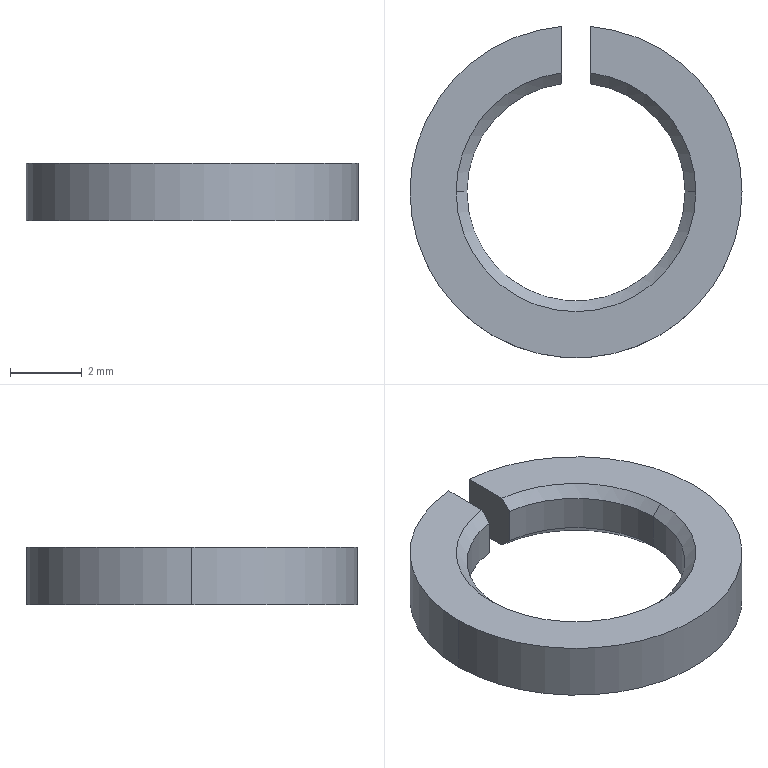Component | SolidWorks | StandardTypeSpringWasher(Assembly)6_1.6[GB_T93-1987]-1 | 1 solid | 16 faces | box 9.28 x 9.26 x 1.6 mm | volume 58 mm3 | cone 6 | cylinder 6 | plane 4 | commonest cylinder face diameters 6.1 x3 9.282 x3
build123d program:
from build123d import *

# Parameters (mm, degrees)
EXTRUDE1_DEPTH = 1.6
CHAMFER1_SIZE  = 0.3


with BuildPart() as part:
    # Sketch1 → Extrude1 (new body)
    with BuildSketch(Plane.XY):
        with BuildLine():
            Line((-0.4, 4.624), (-0.4, 3.024))
            ThreePointArc((-0.4, 3.024), (0, -3.05), (0.4, 3.024))
            Line((0.4, 3.024), (0.4, 4.624))
            ThreePointArc((0.4, 4.624), (0, -4.641), (-0.4, 4.624))
        make_face()
    extrude(amount=EXTRUDE1_DEPTH)

    # Chamfer1
    chamfer1_edges = [part.edges().sort_by_distance(p)[0] for p in [
        (0, -3.05, 1.6),
        (0, -3.05, 0),
    ]]
    chamfer(chamfer1_edges, length=CHAMFER1_SIZE)


solid = part.part

# Placed as in the assembly
solid = solid.moved(Location((120.494, 22.5, 19.6), (0, 0, 0)))
STEP:
#1=COLOUR_RGB('',0.7922,0.8196,0.9333);
#2=FILL_AREA_STYLE_COLOUR('',#1);
#3=FILL_AREA_STYLE('',(#2));
#4=SURFACE_STYLE_FILL_AREA(#3);
#5=SURFACE_SIDE_STYLE('',(#4));
#6=SURFACE_STYLE_USAGE(.BOTH.,#5);
#7=PRESENTATION_STYLE_ASSIGNMENT((#6));
#8=CARTESIAN_POINT('',(4.864,0.8858,0.7835));
#9=VERTEX_POINT('',#8);
#10=CARTESIAN_POINT('',(4.624,0.8858,0.7835));
#11=VERTEX_POINT('',#10);
#12=CARTESIAN_POINT('',(4.744,0.8858,0.7835));
#13=DIRECTION('',(0.,0.,-1.));
#14=DIRECTION('',(1.,0.,0.));
#15=AXIS2_PLACEMENT_3D('',#12,#13,#14);
#16=CIRCLE('',#15,0.1201);
#17=EDGE_CURVE('',#9,#11,#16,.T.);
#18=ORIENTED_EDGE('',*,*,#17,.F.);
#19=CARTESIAN_POINT('',(4.876,0.8858,0.7717));
#20=VERTEX_POINT('',#19);
#21=CARTESIAN_POINT('',(4.864,0.8858,0.7835));
#22=DIRECTION('',(0.7071,0.,-0.7071));
#23=VECTOR('',#22,39.37);
#24=LINE('',#21,#23);
#25=EDGE_CURVE('',#9,#20,#24,.T.);
#26=ORIENTED_EDGE('',*,*,#25,.T.);
#27=CARTESIAN_POINT('',(4.612,0.8858,0.7717));
#28=VERTEX_POINT('',#27);
#29=CARTESIAN_POINT('',(4.744,0.8858,0.7717));
#30=DIRECTION('',(0.,0.,1.));
#31=DIRECTION('',(1.,0.,0.));
#32=AXIS2_PLACEMENT_3D('',#29,#30,#31);
#33=CIRCLE('',#32,0.1319);
#34=EDGE_CURVE('',#28,#20,#33,.T.);
#35=ORIENTED_EDGE('',*,*,#34,.F.);
#36=CARTESIAN_POINT('',(4.624,0.8858,0.7835));
#37=DIRECTION('',(-0.7071,0.,-0.7071));
#38=VECTOR('',#37,39.37);
#39=LINE('',#36,#38);
#40=EDGE_CURVE('',#11,#28,#39,.T.);
#41=ORIENTED_EDGE('',*,*,#40,.F.);
#42=EDGE_LOOP('',(#18,#26,#35,#41));
#43=FACE_OUTER_BOUND('',#42,.T.);
#44=CARTESIAN_POINT('',(4.744,0.8858,0.7835));
#45=DIRECTION('',(0.,0.,-1.));
#46=DIRECTION('',(-1.,0.,0.));
#47=AXIS2_PLACEMENT_3D('',#44,#45,#46);
#48=CONICAL_SURFACE('',#47,0.1201,0.7854);
#49=ADVANCED_FACE('',(#43),#48,.F.);
#50=CARTESIAN_POINT('',(4.728,1.005,0.7835));
#51=VERTEX_POINT('',#50);
#52=CARTESIAN_POINT('',(4.744,0.8858,0.7835));
#53=DIRECTION('',(0.,0.,-1.));
#54=DIRECTION('',(1.,0.,0.));
#55=AXIS2_PLACEMENT_3D('',#52,#53,#54);
#56=CIRCLE('',#55,0.1201);
#57=EDGE_CURVE('',#11,#51,#56,.T.);
#58=ORIENTED_EDGE('',*,*,#57,.F.);
#59=ORIENTED_EDGE('',*,*,#40,.T.);
#60=CARTESIAN_POINT('',(4.728,1.017,0.7717));
#61=VERTEX_POINT('',#60);
#62=CARTESIAN_POINT('',(4.744,0.8858,0.7717));
#63=DIRECTION('',(0.,0.,1.));
#64=DIRECTION('',(1.,0.,0.));
#65=AXIS2_PLACEMENT_3D('',#62,#63,#64);
#66=CIRCLE('',#65,0.1319);
#67=EDGE_CURVE('',#61,#28,#66,.T.);
#68=ORIENTED_EDGE('',*,*,#67,.F.);
#69=CARTESIAN_POINT('',(4.728,1.005,0.7835));
#70=CARTESIAN_POINT('',(4.728,1.009,0.7795));
#71=CARTESIAN_POINT('',(4.728,1.013,0.7756));
#72=CARTESIAN_POINT('',(4.728,1.017,0.7717));
#73=B_SPLINE_CURVE_WITH_KNOTS('',3,(#69,#70,#71,#72),.UNSPECIFIED.,.F.,.F.,(4,4),(0.,0.0004259),.UNSPECIFIED.);
#74=EDGE_CURVE('',#51,#61,#73,.T.);
#75=ORIENTED_EDGE('',*,*,#74,.F.);
#76=EDGE_LOOP('',(#58,#59,#68,#75));
#77=FACE_OUTER_BOUND('',#76,.T.);
#78=CARTESIAN_POINT('',(4.744,0.8858,0.7835));
#79=DIRECTION('',(0.,0.,-1.));
#80=DIRECTION('',(-1.,0.,0.));
#81=AXIS2_PLACEMENT_3D('',#78,#79,#80);
#82=CONICAL_SURFACE('',#81,0.1201,0.7854);
#83=ADVANCED_FACE('',(#77),#82,.F.);
#84=CARTESIAN_POINT('',(4.624,0.8858,0.8228));
#85=VERTEX_POINT('',#84);
#86=CARTESIAN_POINT('',(4.864,0.8858,0.8228));
#87=VERTEX_POINT('',#86);
#88=CARTESIAN_POINT('',(4.744,0.8858,0.8228));
#89=DIRECTION('',(0.,0.,1.));
#90=DIRECTION('',(1.,0.,0.));
#91=AXIS2_PLACEMENT_3D('',#88,#89,#90);
#92=CIRCLE('',#91,0.1201);
#93=EDGE_CURVE('',#85,#87,#92,.T.);
#94=ORIENTED_EDGE('',*,*,#93,.F.);
#95=CARTESIAN_POINT('',(4.612,0.8858,0.8346));
#96=VERTEX_POINT('',#95);
#97=CARTESIAN_POINT('',(4.612,0.8858,0.8346));
#98=DIRECTION('',(-0.7071,0.,0.7071));
#99=VECTOR('',#98,39.37);
#100=LINE('',#97,#99);
#101=EDGE_CURVE('',#85,#96,#100,.T.);
#102=ORIENTED_EDGE('',*,*,#101,.T.);
#103=CARTESIAN_POINT('',(4.876,0.8858,0.8346));
#104=VERTEX_POINT('',#103);
#105=CARTESIAN_POINT('',(4.744,0.8858,0.8346));
#106=DIRECTION('',(0.,0.,-1.));
#107=DIRECTION('',(1.,0.,0.));
#108=AXIS2_PLACEMENT_3D('',#105,#106,#107);
#109=CIRCLE('',#108,0.1319);
#110=EDGE_CURVE('',#104,#96,#109,.T.);
#111=ORIENTED_EDGE('',*,*,#110,.F.);
#112=CARTESIAN_POINT('',(4.876,0.8858,0.8346));
#113=DIRECTION('',(0.7071,0.,0.7071));
#114=VECTOR('',#113,39.37);
#115=LINE('',#112,#114);
#116=EDGE_CURVE('',#87,#104,#115,.T.);
#117=ORIENTED_EDGE('',*,*,#116,.F.);
#118=EDGE_LOOP('',(#94,#102,#111,#117));
#119=FACE_OUTER_BOUND('',#118,.T.);
#120=CARTESIAN_POINT('',(4.744,0.8858,0.8346));
#121=DIRECTION('',(0.,0.,1.));
#122=DIRECTION('',(1.,0.,0.));
#123=AXIS2_PLACEMENT_3D('',#120,#121,#122);
#124=CONICAL_SURFACE('',#123,0.1319,0.7854);
#125=ADVANCED_FACE('',(#119),#124,.F.);
#126=CARTESIAN_POINT('',(4.76,1.005,0.8228));
#127=VERTEX_POINT('',#126);
#128=CARTESIAN_POINT('',(4.744,0.8858,0.8228));
#129=DIRECTION('',(0.,0.,1.));
#130=DIRECTION('',(1.,0.,0.));
#131=AXIS2_PLACEMENT_3D('',#128,#129,#130);
#132=CIRCLE('',#131,0.1201);
#133=EDGE_CURVE('',#87,#127,#132,.T.);
#134=ORIENTED_EDGE('',*,*,#133,.F.);
#135=ORIENTED_EDGE('',*,*,#116,.T.);
#136=CARTESIAN_POINT('',(4.76,1.017,0.8346));
#137=VERTEX_POINT('',#136);
#138=CARTESIAN_POINT('',(4.744,0.8858,0.8346));
#139=DIRECTION('',(0.,0.,-1.));
#140=DIRECTION('',(1.,0.,0.));
#141=AXIS2_PLACEMENT_3D('',#138,#139,#140);
#142=CIRCLE('',#141,0.1319);
#143=EDGE_CURVE('',#137,#104,#142,.T.);
#144=ORIENTED_EDGE('',*,*,#143,.F.);
#145=CARTESIAN_POINT('',(4.76,1.005,0.8228));
#146=CARTESIAN_POINT('',(4.76,1.009,0.8268));
#147=CARTESIAN_POINT('',(4.76,1.013,0.8307));
#148=CARTESIAN_POINT('',(4.76,1.017,0.8346));
#149=B_SPLINE_CURVE_WITH_KNOTS('',3,(#145,#146,#147,#148),.UNSPECIFIED.,.F.,.F.,(4,4),(0.,0.0004259),.UNSPECIFIED.);
#150=EDGE_CURVE('',#127,#137,#149,.T.);
#151=ORIENTED_EDGE('',*,*,#150,.F.);
#152=EDGE_LOOP('',(#134,#135,#144,#151));
#153=FACE_OUTER_BOUND('',#152,.T.);
#154=CARTESIAN_POINT('',(4.744,0.8858,0.8346));
#155=DIRECTION('',(0.,0.,1.));
#156=DIRECTION('',(1.,0.,0.));
#157=AXIS2_PLACEMENT_3D('',#154,#155,#156);
#158=CONICAL_SURFACE('',#157,0.1319,0.7854);
#159=ADVANCED_FACE('',(#153),#158,.F.);
#160=ORIENTED_EDGE('',*,*,#93,.T.);
#161=CARTESIAN_POINT('',(4.864,0.8858,0.8346));
#162=DIRECTION('',(0.,0.,-1.));
#163=VECTOR('',#162,39.37);
#164=LINE('',#161,#163);
#165=EDGE_CURVE('',#87,#9,#164,.T.);
#166=ORIENTED_EDGE('',*,*,#165,.T.);
#167=ORIENTED_EDGE('',*,*,#17,.T.);
#168=CARTESIAN_POINT('',(4.624,0.8858,0.8346));
#169=DIRECTION('',(0.,0.,-1.));
#170=VECTOR('',#169,39.37);
#171=LINE('',#168,#170);
#172=EDGE_CURVE('',#85,#11,#171,.T.);
#173=ORIENTED_EDGE('',*,*,#172,.F.);
#174=EDGE_LOOP('',(#160,#166,#167,#173));
#175=FACE_OUTER_BOUND('',#174,.T.);
#176=CARTESIAN_POINT('',(4.744,0.8858,0.8346));
#177=DIRECTION('',(0.,0.,-1.));
#178=DIRECTION('',(-1.,0.,0.));
#179=AXIS2_PLACEMENT_3D('',#176,#177,#178);
#180=CYLINDRICAL_SURFACE('',#179,0.1201);
#181=ADVANCED_FACE('',(#175),#180,.F.);
#182=CARTESIAN_POINT('',(4.728,1.005,0.8228));
#183=VERTEX_POINT('',#182);
#184=CARTESIAN_POINT('',(4.744,0.8858,0.8228));
#185=DIRECTION('',(0.,0.,1.));
#186=DIRECTION('',(1.,0.,0.));
#187=AXIS2_PLACEMENT_3D('',#184,#185,#186);
#188=CIRCLE('',#187,0.1201);
#189=EDGE_CURVE('',#183,#85,#188,.T.);
#190=ORIENTED_EDGE('',*,*,#189,.T.);
#191=ORIENTED_EDGE('',*,*,#172,.T.);
#192=ORIENTED_EDGE('',*,*,#57,.T.);
#193=CARTESIAN_POINT('',(4.728,1.005,0.8346));
#194=DIRECTION('',(0.,0.,-1.));
#195=VECTOR('',#194,39.37);
#196=LINE('',#193,#195);
#197=EDGE_CURVE('',#183,#51,#196,.T.);
#198=ORIENTED_EDGE('',*,*,#197,.F.);
#199=EDGE_LOOP('',(#190,#191,#192,#198));
#200=FACE_OUTER_BOUND('',#199,.T.);
#201=CARTESIAN_POINT('',(4.744,0.8858,0.8346));
#202=DIRECTION('',(0.,0.,-1.));
#203=DIRECTION('',(-1.,0.,0.));
#204=AXIS2_PLACEMENT_3D('',#201,#202,#203);
#205=CYLINDRICAL_SURFACE('',#204,0.1201);
#206=ADVANCED_FACE('',(#200),#205,.F.);
#207=CARTESIAN_POINT('',(4.927,0.8858,0.8346));
#208=VERTEX_POINT('',#207);
#209=CARTESIAN_POINT('',(4.76,1.068,0.8346));
#210=VERTEX_POINT('',#209);
#211=CARTESIAN_POINT('',(4.744,0.8858,0.8346));
#212=DIRECTION('',(0.,0.,1.));
#213=DIRECTION('',(1.,0.,0.));
#214=AXIS2_PLACEMENT_3D('',#211,#212,#213);
#215=CIRCLE('',#214,0.1827);
#216=EDGE_CURVE('',#208,#210,#215,.T.);
#217=ORIENTED_EDGE('',*,*,#216,.F.);
#218=CARTESIAN_POINT('',(4.927,0.8858,0.7717));
#219=VERTEX_POINT('',#218);
#220=CARTESIAN_POINT('',(4.927,0.8858,0.8346));
#221=DIRECTION('',(0.,0.,-1.));
#222=VECTOR('',#221,39.37);
#223=LINE('',#220,#222);
#224=EDGE_CURVE('',#208,#219,#223,.T.);
#225=ORIENTED_EDGE('',*,*,#224,.T.);
#226=CARTESIAN_POINT('',(4.76,1.068,0.7717));
#227=VERTEX_POINT('',#226);
#228=CARTESIAN_POINT('',(4.744,0.8858,0.7717));
#229=DIRECTION('',(0.,0.,1.));
#230=DIRECTION('',(1.,0.,0.));
#231=AXIS2_PLACEMENT_3D('',#228,#229,#230);
#232=CIRCLE('',#231,0.1827);
#233=EDGE_CURVE('',#219,#227,#232,.T.);
#234=ORIENTED_EDGE('',*,*,#233,.T.);
#235=CARTESIAN_POINT('',(4.76,1.068,0.8346));
#236=DIRECTION('',(0.,0.,-1.));
#237=VECTOR('',#236,39.37);
#238=LINE('',#235,#237);
#239=EDGE_CURVE('',#210,#227,#238,.T.);
#240=ORIENTED_EDGE('',*,*,#239,.F.);
#241=EDGE_LOOP('',(#217,#225,#234,#240));
#242=FACE_OUTER_BOUND('',#241,.T.);
#243=CARTESIAN_POINT('',(4.744,0.8858,0.8346));
#244=DIRECTION('',(0.,0.,-1.));
#245=DIRECTION('',(-1.,0.,0.));
#246=AXIS2_PLACEMENT_3D('',#243,#244,#245);
#247=CYLINDRICAL_SURFACE('',#246,0.1827);
#248=ADVANCED_FACE('',(#242),#247,.T.);
#249=ORIENTED_EDGE('',*,*,#224,.F.);
#250=CARTESIAN_POINT('',(4.561,0.8858,0.8346));
#251=VERTEX_POINT('',#250);
#252=CARTESIAN_POINT('',(4.744,0.8858,0.8346));
#253=DIRECTION('',(0.,0.,1.));
#254=DIRECTION('',(1.,0.,0.));
#255=AXIS2_PLACEMENT_3D('',#252,#253,#254);
#256=CIRCLE('',#255,0.1827);
#257=EDGE_CURVE('',#251,#208,#256,.T.);
#258=ORIENTED_EDGE('',*,*,#257,.F.);
#259=CARTESIAN_POINT('',(4.561,0.8858,0.7717));
#260=VERTEX_POINT('',#259);
#261=CARTESIAN_POINT('',(4.561,0.8858,0.8346));
#262=DIRECTION('',(0.,0.,-1.));
#263=VECTOR('',#262,39.37);
#264=LINE('',#261,#263);
#265=EDGE_CURVE('',#251,#260,#264,.T.);
#266=ORIENTED_EDGE('',*,*,#265,.T.);
#267=CARTESIAN_POINT('',(4.744,0.8858,0.7717));
#268=DIRECTION('',(0.,0.,1.));
#269=DIRECTION('',(1.,0.,0.));
#270=AXIS2_PLACEMENT_3D('',#267,#268,#269);
#271=CIRCLE('',#270,0.1827);
#272=EDGE_CURVE('',#260,#219,#271,.T.);
#273=ORIENTED_EDGE('',*,*,#272,.T.);
#274=EDGE_LOOP('',(#249,#258,#266,#273));
#275=FACE_OUTER_BOUND('',#274,.T.);
#276=CARTESIAN_POINT('',(4.744,0.8858,0.8346));
#277=DIRECTION('',(0.,0.,-1.));
#278=DIRECTION('',(-1.,0.,0.));
#279=AXIS2_PLACEMENT_3D('',#276,#277,#278);
#280=CYLINDRICAL_SURFACE('',#279,0.1827);
#281=ADVANCED_FACE('',(#275),#280,.T.);
#282=ORIENTED_EDGE('',*,*,#265,.F.);
#283=CARTESIAN_POINT('',(4.728,1.068,0.8346));
#284=VERTEX_POINT('',#283);
#285=CARTESIAN_POINT('',(4.744,0.8858,0.8346));
#286=DIRECTION('',(0.,0.,1.));
#287=DIRECTION('',(1.,0.,0.));
#288=AXIS2_PLACEMENT_3D('',#285,#286,#287);
#289=CIRCLE('',#288,0.1827);
#290=EDGE_CURVE('',#284,#251,#289,.T.);
#291=ORIENTED_EDGE('',*,*,#290,.F.);
#292=CARTESIAN_POINT('',(4.728,1.068,0.7717));
#293=VERTEX_POINT('',#292);
#294=CARTESIAN_POINT('',(4.728,1.068,0.8346));
#295=DIRECTION('',(0.,0.,-1.));
#296=VECTOR('',#295,39.37);
#297=LINE('',#294,#296);
#298=EDGE_CURVE('',#284,#293,#297,.T.);
#299=ORIENTED_EDGE('',*,*,#298,.T.);
#300=CARTESIAN_POINT('',(4.744,0.8858,0.7717));
#301=DIRECTION('',(0.,0.,1.));
#302=DIRECTION('',(1.,0.,0.));
#303=AXIS2_PLACEMENT_3D('',#300,#301,#302);
#304=CIRCLE('',#303,0.1827);
#305=EDGE_CURVE('',#293,#260,#304,.T.);
#306=ORIENTED_EDGE('',*,*,#305,.T.);
#307=EDGE_LOOP('',(#282,#291,#299,#306));
#308=FACE_OUTER_BOUND('',#307,.T.);
#309=CARTESIAN_POINT('',(4.744,0.8858,0.8346));
#310=DIRECTION('',(0.,0.,-1.));
#311=DIRECTION('',(-1.,0.,0.));
#312=AXIS2_PLACEMENT_3D('',#309,#310,#311);
#313=CYLINDRICAL_SURFACE('',#312,0.1827);
#314=ADVANCED_FACE('',(#308),#313,.T.);
#315=CARTESIAN_POINT('',(4.76,1.005,0.7835));
#316=VERTEX_POINT('',#315);
#317=CARTESIAN_POINT('',(4.76,1.005,0.8346));
#318=DIRECTION('',(0.,0.,-1.));
#319=VECTOR('',#318,39.37);
#320=LINE('',#317,#319);
#321=EDGE_CURVE('',#127,#316,#320,.T.);
#322=ORIENTED_EDGE('',*,*,#321,.F.);
#323=ORIENTED_EDGE('',*,*,#150,.T.);
#324=CARTESIAN_POINT('',(4.76,1.068,0.8346));
#325=DIRECTION('',(0.,-1.,0.));
#326=VECTOR('',#325,39.37);
#327=LINE('',#324,#326);
#328=EDGE_CURVE('',#210,#137,#327,.T.);
#329=ORIENTED_EDGE('',*,*,#328,.F.);
#330=ORIENTED_EDGE('',*,*,#239,.T.);
#331=CARTESIAN_POINT('',(4.76,1.017,0.7717));
#332=VERTEX_POINT('',#331);
#333=CARTESIAN_POINT('',(4.76,1.068,0.7717));
#334=DIRECTION('',(0.,-1.,0.));
#335=VECTOR('',#334,39.37);
#336=LINE('',#333,#335);
#337=EDGE_CURVE('',#227,#332,#336,.T.);
#338=ORIENTED_EDGE('',*,*,#337,.T.);
#339=CARTESIAN_POINT('',(4.76,1.017,0.7717));
#340=CARTESIAN_POINT('',(4.76,1.013,0.7756));
#341=CARTESIAN_POINT('',(4.76,1.009,0.7795));
#342=CARTESIAN_POINT('',(4.76,1.005,0.7835));
#343=B_SPLINE_CURVE_WITH_KNOTS('',3,(#339,#340,#341,#342),.UNSPECIFIED.,.F.,.F.,(4,4),(0.,0.0004259),.UNSPECIFIED.);
#344=EDGE_CURVE('',#332,#316,#343,.T.);
#345=ORIENTED_EDGE('',*,*,#344,.T.);
#346=EDGE_LOOP('',(#322,#323,#329,#330,#338,#345));
#347=FACE_OUTER_BOUND('',#346,.T.);
#348=CARTESIAN_POINT('',(4.76,1.068,0.8346));
#349=DIRECTION('',(1.,0.,0.));
#350=DIRECTION('',(-0.,1.,0.));
#351=AXIS2_PLACEMENT_3D('',#348,#349,#350);
#352=PLANE('',#351);
#353=ADVANCED_FACE('',(#347),#352,.F.);
#354=ORIENTED_EDGE('',*,*,#165,.F.);
#355=ORIENTED_EDGE('',*,*,#133,.T.);
#356=ORIENTED_EDGE('',*,*,#321,.T.);
#357=CARTESIAN_POINT('',(4.744,0.8858,0.7835));
#358=DIRECTION('',(0.,0.,-1.));
#359=DIRECTION('',(1.,0.,0.));
#360=AXIS2_PLACEMENT_3D('',#357,#358,#359);
#361=CIRCLE('',#360,0.1201);
#362=EDGE_CURVE('',#316,#9,#361,.T.);
#363=ORIENTED_EDGE('',*,*,#362,.T.);
#364=EDGE_LOOP('',(#354,#355,#356,#363));
#365=FACE_OUTER_BOUND('',#364,.T.);
#366=CARTESIAN_POINT('',(4.744,0.8858,0.8346));
#367=DIRECTION('',(0.,0.,-1.));
#368=DIRECTION('',(-1.,0.,0.));
#369=AXIS2_PLACEMENT_3D('',#366,#367,#368);
#370=CYLINDRICAL_SURFACE('',#369,0.1201);
#371=ADVANCED_FACE('',(#365),#370,.F.);
#372=CARTESIAN_POINT('',(4.728,1.017,0.8346));
#373=VERTEX_POINT('',#372);
#374=CARTESIAN_POINT('',(4.728,1.068,0.8346));
#375=DIRECTION('',(0.,1.,0.));
#376=VECTOR('',#375,39.37);
#377=LINE('',#374,#376);
#378=EDGE_CURVE('',#373,#284,#377,.T.);
#379=ORIENTED_EDGE('',*,*,#378,.F.);
#380=CARTESIAN_POINT('',(4.728,1.017,0.8346));
#381=CARTESIAN_POINT('',(4.728,1.013,0.8307));
#382=CARTESIAN_POINT('',(4.728,1.009,0.8268));
#383=CARTESIAN_POINT('',(4.728,1.005,0.8228));
#384=B_SPLINE_CURVE_WITH_KNOTS('',3,(#380,#381,#382,#383),.UNSPECIFIED.,.F.,.F.,(4,4),(0.,0.0004259),.UNSPECIFIED.);
#385=EDGE_CURVE('',#373,#183,#384,.T.);
#386=ORIENTED_EDGE('',*,*,#385,.T.);
#387=ORIENTED_EDGE('',*,*,#197,.T.);
#388=ORIENTED_EDGE('',*,*,#74,.T.);
#389=CARTESIAN_POINT('',(4.728,1.068,0.7717));
#390=DIRECTION('',(0.,1.,0.));
#391=VECTOR('',#390,39.37);
#392=LINE('',#389,#391);
#393=EDGE_CURVE('',#61,#293,#392,.T.);
#394=ORIENTED_EDGE('',*,*,#393,.T.);
#395=ORIENTED_EDGE('',*,*,#298,.F.);
#396=EDGE_LOOP('',(#379,#386,#387,#388,#394,#395));
#397=FACE_OUTER_BOUND('',#396,.T.);
#398=CARTESIAN_POINT('',(4.728,1.068,0.8346));
#399=DIRECTION('',(-1.,0.,0.));
#400=DIRECTION('',(0.,0.,1.));
#401=AXIS2_PLACEMENT_3D('',#398,#399,#400);
#402=PLANE('',#401);
#403=ADVANCED_FACE('',(#397),#402,.F.);
#404=ORIENTED_EDGE('',*,*,#328,.T.);
#405=ORIENTED_EDGE('',*,*,#143,.T.);
#406=ORIENTED_EDGE('',*,*,#110,.T.);
#407=CARTESIAN_POINT('',(4.744,0.8858,0.8346));
#408=DIRECTION('',(0.,0.,-1.));
#409=DIRECTION('',(1.,0.,0.));
#410=AXIS2_PLACEMENT_3D('',#407,#408,#409);
#411=CIRCLE('',#410,0.1319);
#412=EDGE_CURVE('',#96,#373,#411,.T.);
#413=ORIENTED_EDGE('',*,*,#412,.T.);
#414=ORIENTED_EDGE('',*,*,#378,.T.);
#415=ORIENTED_EDGE('',*,*,#290,.T.);
#416=ORIENTED_EDGE('',*,*,#257,.T.);
#417=ORIENTED_EDGE('',*,*,#216,.T.);
#418=EDGE_LOOP('',(#404,#405,#406,#413,#414,#415,#416,#417));
#419=FACE_OUTER_BOUND('',#418,.T.);
#420=CARTESIAN_POINT('',(4.744,0.8858,0.8346));
#421=DIRECTION('',(0.,0.,1.));
#422=DIRECTION('',(1.,0.,0.));
#423=AXIS2_PLACEMENT_3D('',#420,#421,#422);
#424=PLANE('',#423);
#425=ADVANCED_FACE('',(#419),#424,.T.);
#426=ORIENTED_EDGE('',*,*,#393,.F.);
#427=ORIENTED_EDGE('',*,*,#67,.T.);
#428=ORIENTED_EDGE('',*,*,#34,.T.);
#429=CARTESIAN_POINT('',(4.744,0.8858,0.7717));
#430=DIRECTION('',(0.,0.,1.));
#431=DIRECTION('',(1.,0.,0.));
#432=AXIS2_PLACEMENT_3D('',#429,#430,#431);
#433=CIRCLE('',#432,0.1319);
#434=EDGE_CURVE('',#20,#332,#433,.T.);
#435=ORIENTED_EDGE('',*,*,#434,.T.);
#436=ORIENTED_EDGE('',*,*,#337,.F.);
#437=ORIENTED_EDGE('',*,*,#233,.F.);
#438=ORIENTED_EDGE('',*,*,#272,.F.);
#439=ORIENTED_EDGE('',*,*,#305,.F.);
#440=EDGE_LOOP('',(#426,#427,#428,#435,#436,#437,#438,#439));
#441=FACE_OUTER_BOUND('',#440,.T.);
#442=CARTESIAN_POINT('',(4.744,0.8858,0.7717));
#443=DIRECTION('',(0.,0.,1.));
#444=DIRECTION('',(1.,0.,0.));
#445=AXIS2_PLACEMENT_3D('',#442,#443,#444);
#446=PLANE('',#445);
#447=ADVANCED_FACE('',(#441),#446,.F.);
#448=ORIENTED_EDGE('',*,*,#101,.F.);
#449=ORIENTED_EDGE('',*,*,#189,.F.);
#450=ORIENTED_EDGE('',*,*,#385,.F.);
#451=ORIENTED_EDGE('',*,*,#412,.F.);
#452=EDGE_LOOP('',(#448,#449,#450,#451));
#453=FACE_OUTER_BOUND('',#452,.T.);
#454=CARTESIAN_POINT('',(4.744,0.8858,0.8346));
#455=DIRECTION('',(0.,0.,1.));
#456=DIRECTION('',(1.,0.,0.));
#457=AXIS2_PLACEMENT_3D('',#454,#455,#456);
#458=CONICAL_SURFACE('',#457,0.1319,0.7854);
#459=ADVANCED_FACE('',(#453),#458,.F.);
#460=ORIENTED_EDGE('',*,*,#25,.F.);
#461=ORIENTED_EDGE('',*,*,#362,.F.);
#462=ORIENTED_EDGE('',*,*,#344,.F.);
#463=ORIENTED_EDGE('',*,*,#434,.F.);
#464=EDGE_LOOP('',(#460,#461,#462,#463));
#465=FACE_OUTER_BOUND('',#464,.T.);
#466=CARTESIAN_POINT('',(4.744,0.8858,0.7835));
#467=DIRECTION('',(0.,0.,-1.));
#468=DIRECTION('',(-1.,0.,0.));
#469=AXIS2_PLACEMENT_3D('',#466,#467,#468);
#470=CONICAL_SURFACE('',#469,0.1201,0.7854);
#471=ADVANCED_FACE('',(#465),#470,.F.);
#472=CLOSED_SHELL('',(#49,#83,#125,#159,#181,#206,#248,#281,#314,#353,#371,#403,#425,#447,#459,#471));
#473=MANIFOLD_SOLID_BREP('',#472);
#474=STYLED_ITEM('',(#7),#473);
#475=PRESENTATION_LAYER_ASSIGNMENT('','',(#474));
#476=(LENGTH_UNIT()NAMED_UNIT(*)SI_UNIT($,.METRE.));
#477=LENGTH_MEASURE_WITH_UNIT(LENGTH_MEASURE(0.0254),#476);
#478=DIMENSIONAL_EXPONENTS(1.,0.,0.,0.,0.,0.,0.);
#479=(CONVERSION_BASED_UNIT('',#477)LENGTH_UNIT()NAMED_UNIT(#478));
#480=UNCERTAINTY_MEASURE_WITH_UNIT(LENGTH_MEASURE(0.00001),#479,'','');
#481=(NAMED_UNIT(*)PLANE_ANGLE_UNIT()SI_UNIT($,.RADIAN.));
#482=(NAMED_UNIT(*)SI_UNIT($,.STERADIAN.)SOLID_ANGLE_UNIT());
#483=(GEOMETRIC_REPRESENTATION_CONTEXT(3)GLOBAL_UNCERTAINTY_ASSIGNED_CONTEXT((#480))GLOBAL_UNIT_ASSIGNED_CONTEXT((#479,#481,#482))REPRESENTATION_CONTEXT('',''));
#484=MECHANICAL_DESIGN_GEOMETRIC_PRESENTATION_REPRESENTATION('',(#474),#483);
#485=CARTESIAN_POINT('',(0.,0.,0.));
#486=DIRECTION('',(0.,0.,1.));
#487=DIRECTION('',(1.,0.,0.));
#488=AXIS2_PLACEMENT_3D('',#485,#486,#487);
#489=(LENGTH_UNIT()NAMED_UNIT(*)SI_UNIT($,.METRE.));
#490=LENGTH_MEASURE_WITH_UNIT(LENGTH_MEASURE(0.0254),#489);
#491=DIMENSIONAL_EXPONENTS(1.,0.,0.,0.,0.,0.,0.);
#492=(CONVERSION_BASED_UNIT('',#490)LENGTH_UNIT()NAMED_UNIT(#491));
#493=UNCERTAINTY_MEASURE_WITH_UNIT(LENGTH_MEASURE(0.00001),#492,'','');
#494=(NAMED_UNIT(*)PLANE_ANGLE_UNIT()SI_UNIT($,.RADIAN.));
#495=(NAMED_UNIT(*)SI_UNIT($,.STERADIAN.)SOLID_ANGLE_UNIT());
#496=(GEOMETRIC_REPRESENTATION_CONTEXT(3)GLOBAL_UNCERTAINTY_ASSIGNED_CONTEXT((#493))GLOBAL_UNIT_ASSIGNED_CONTEXT((#492,#494,#495))REPRESENTATION_CONTEXT('',''));
#497=ADVANCED_BREP_SHAPE_REPRESENTATION('',(#473,#488),#496);